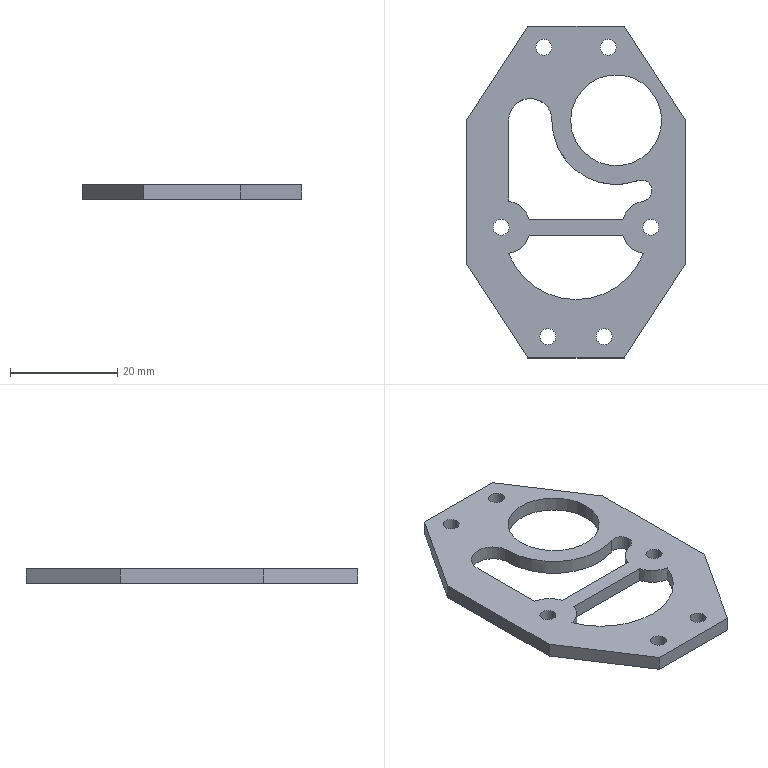Component | NX | BASE-PLATE | 1 solid | 28 faces | volume 3614 mm3 | plane 13 | cylinder 13 | other 2 | commonest cylinder face diameters 3 x6 10 x4 3.936 x1 27 x1 17 x1